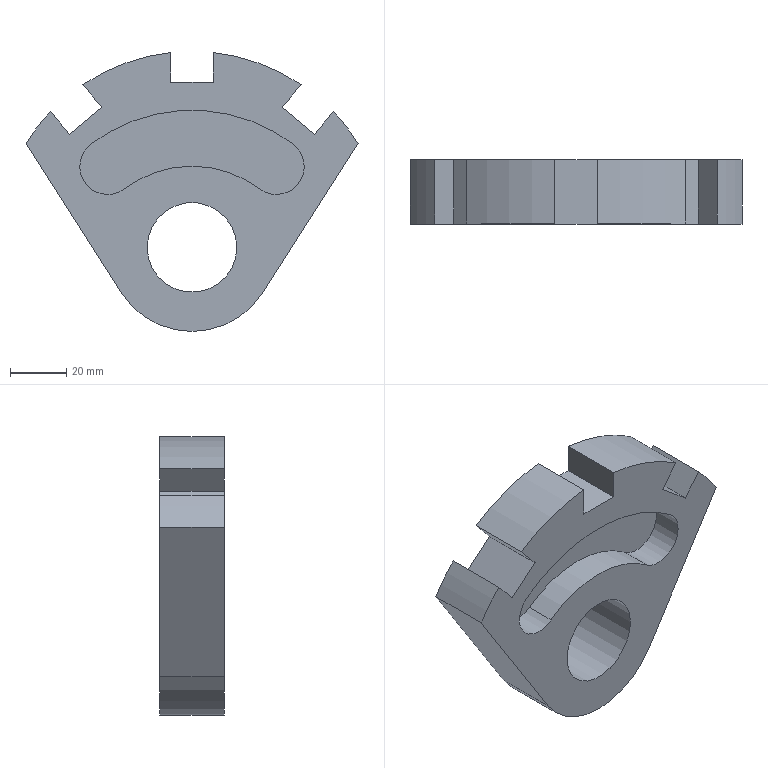Component | NX | SECTOR_PART | 1 solid | 24 faces | volume 130850 mm3 | plane 14 | cylinder 10 | commonest cylinder face diameters 140 x4 20 x2 60 x1 32 x1 80 x1 120 x1